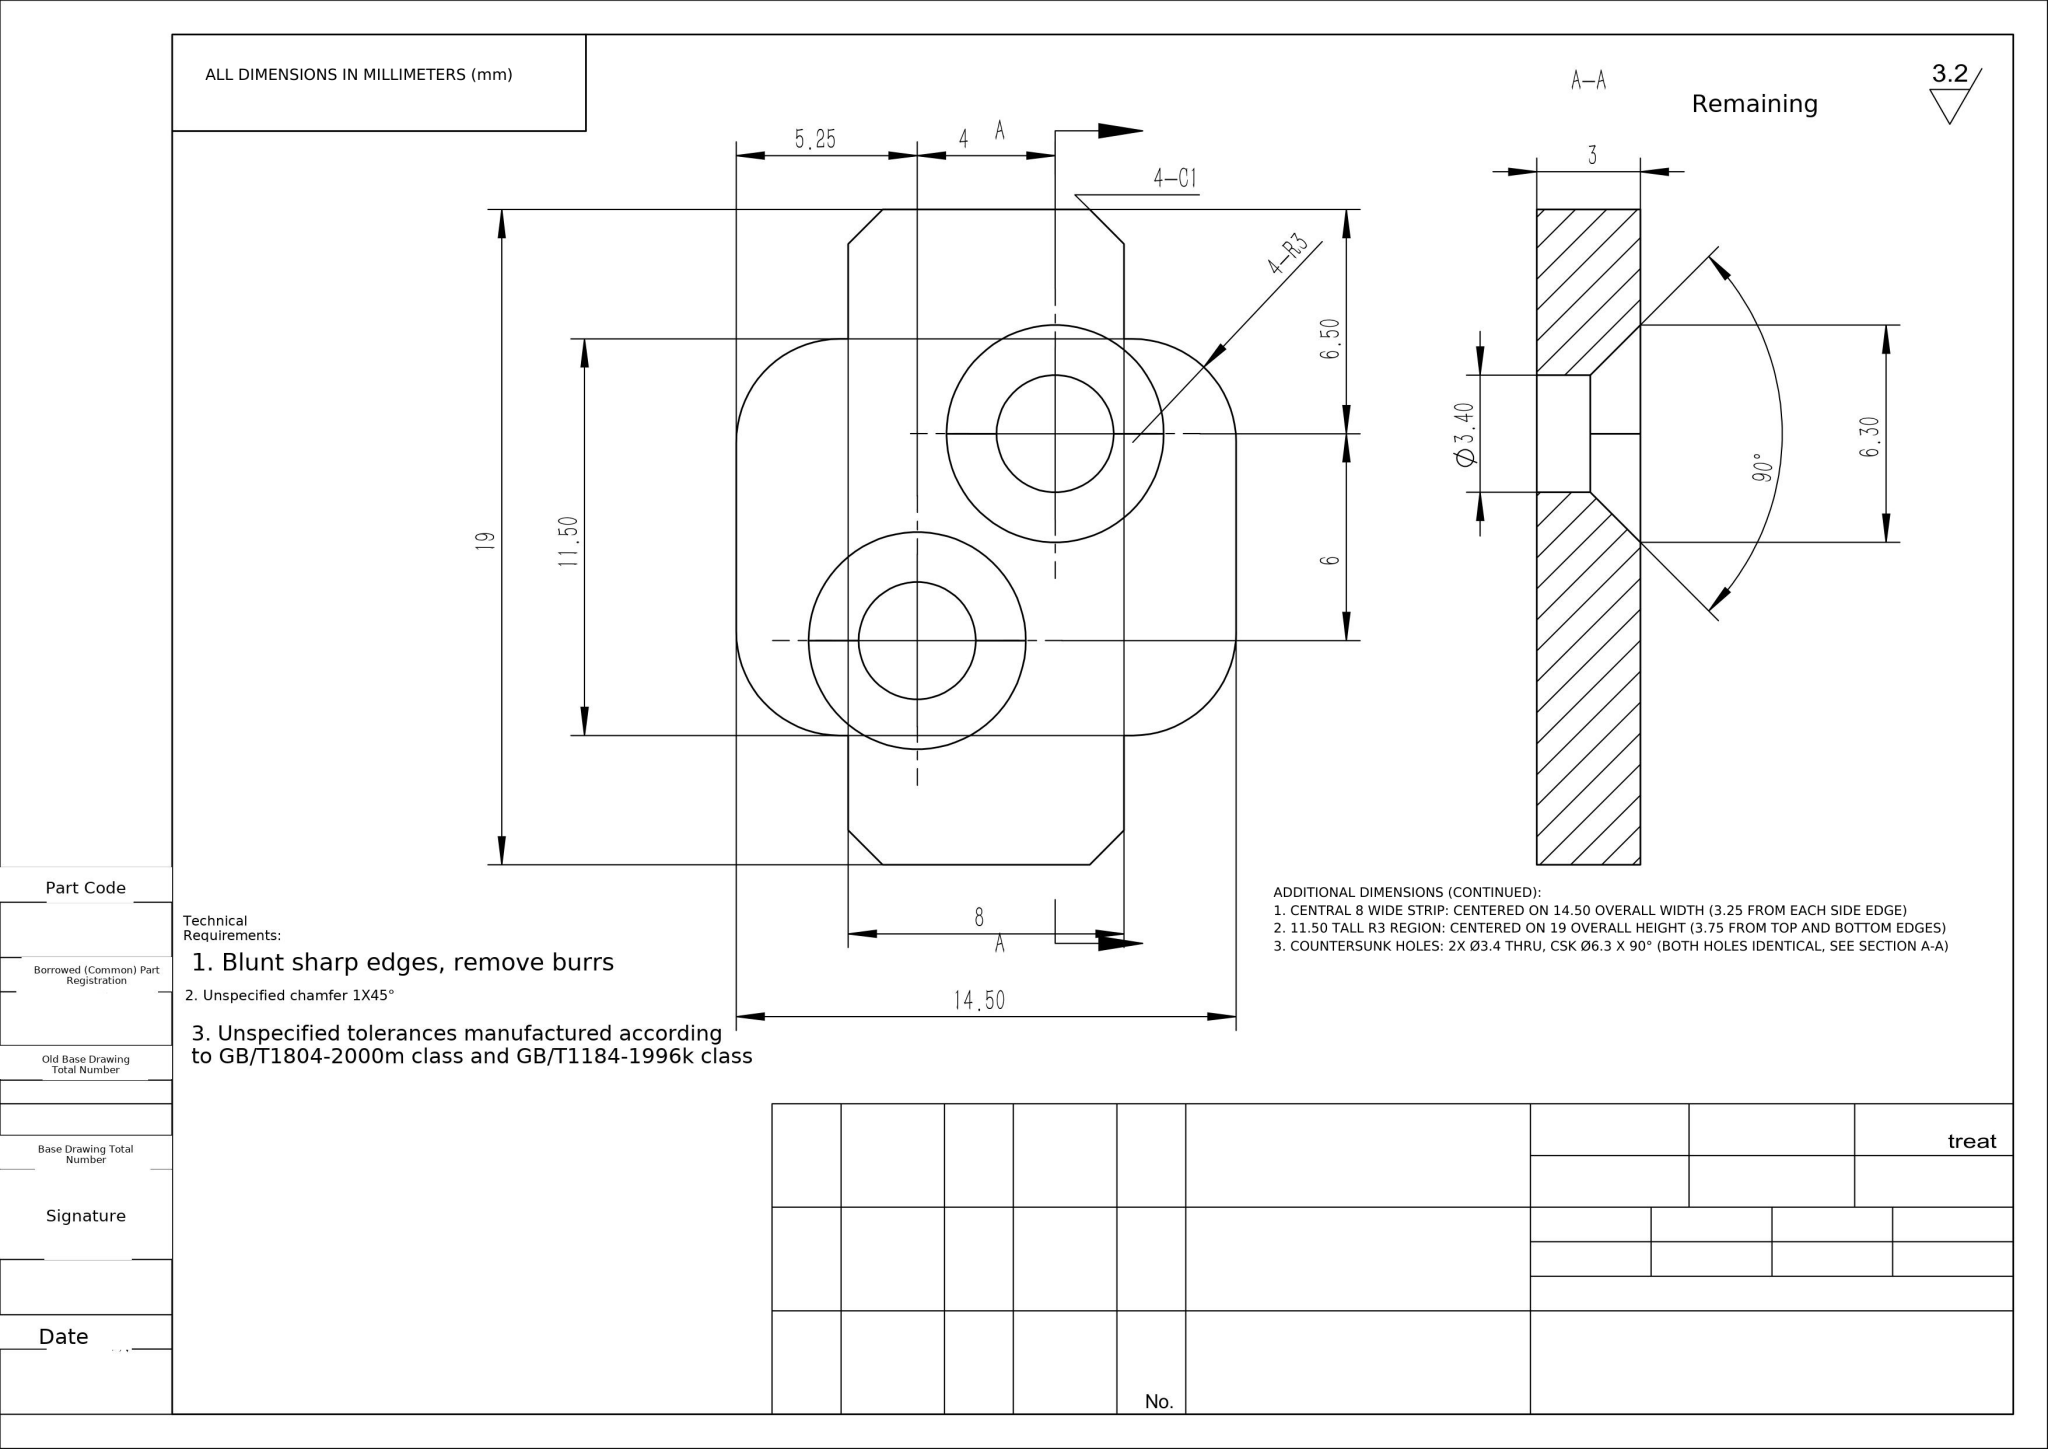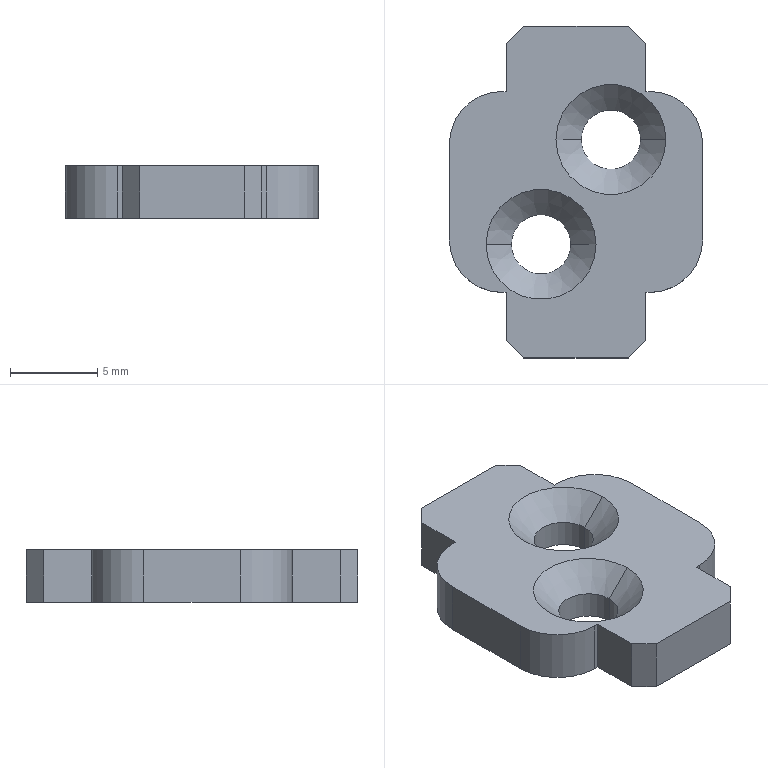Part | NX | mm | 1 solid | 30 faces | box 14.5 x 19 x 3 mm | volume 568 mm3 | plane 18 | cylinder 8 | cone 4 | commonest cylinder face diameters 3.4 x4 6 x4
STEP:
#1=COLOUR_RGB('',1.,1.,1.);
#2=FILL_AREA_STYLE_COLOUR('',#1);
#3=FILL_AREA_STYLE('',(#2));
#4=SURFACE_STYLE_FILL_AREA(#3);
#5=SURFACE_SIDE_STYLE('',(#4));
#6=SURFACE_STYLE_USAGE(.BOTH.,#5);
#7=PRESENTATION_STYLE_ASSIGNMENT((#6));
#8=CARTESIAN_POINT('',(-0.3,-3.,-1.5));
#9=VERTEX_POINT('',#8);
#10=CARTESIAN_POINT('',(-3.7,-3.,-1.5));
#11=VERTEX_POINT('',#10);
#12=CARTESIAN_POINT('',(-2.,-3.,-1.5));
#13=DIRECTION('',(0.,0.,-1.));
#14=DIRECTION('',(1.,0.,0.));
#15=AXIS2_PLACEMENT_3D('',#12,#13,#14);
#16=CIRCLE('',#15,1.7);
#17=EDGE_CURVE('',#9,#11,#16,.T.);
#18=ORIENTED_EDGE('',*,*,#17,.T.);
#19=CARTESIAN_POINT('',(-3.7,-3.,0.05));
#20=VERTEX_POINT('',#19);
#21=CARTESIAN_POINT('',(-3.7,-3.,-22.588));
#22=DIRECTION('',(0.,0.,1.));
#23=VECTOR('',#22,1000.);
#24=LINE('',#21,#23);
#25=EDGE_CURVE('',#11,#20,#24,.T.);
#26=ORIENTED_EDGE('',*,*,#25,.T.);
#27=CARTESIAN_POINT('',(-0.3,-3.,0.05));
#28=VERTEX_POINT('',#27);
#29=CARTESIAN_POINT('',(-2.,-3.,0.05));
#30=DIRECTION('',(0.,0.,-1.));
#31=DIRECTION('',(1.,0.,0.));
#32=AXIS2_PLACEMENT_3D('',#29,#30,#31);
#33=CIRCLE('',#32,1.7);
#34=EDGE_CURVE('',#28,#20,#33,.T.);
#35=ORIENTED_EDGE('',*,*,#34,.F.);
#36=CARTESIAN_POINT('',(-0.3,-3.,-22.588));
#37=DIRECTION('',(0.,0.,1.));
#38=VECTOR('',#37,1000.);
#39=LINE('',#36,#38);
#40=EDGE_CURVE('',#9,#28,#39,.T.);
#41=ORIENTED_EDGE('',*,*,#40,.F.);
#42=EDGE_LOOP('',(#18,#26,#35,#41));
#43=FACE_OUTER_BOUND('',#42,.T.);
#44=CARTESIAN_POINT('',(-2.,-3.,-22.588));
#45=DIRECTION('',(0.,0.,1.));
#46=DIRECTION('',(1.,0.,0.));
#47=AXIS2_PLACEMENT_3D('',#44,#45,#46);
#48=CYLINDRICAL_SURFACE('',#47,1.7);
#49=ADVANCED_FACE('',(#43),#48,.F.);
#50=CARTESIAN_POINT('',(3.7,3.,-1.5));
#51=VERTEX_POINT('',#50);
#52=CARTESIAN_POINT('',(0.3,3.,-1.5));
#53=VERTEX_POINT('',#52);
#54=CARTESIAN_POINT('',(2.,3.,-1.5));
#55=DIRECTION('',(0.,0.,-1.));
#56=DIRECTION('',(1.,0.,0.));
#57=AXIS2_PLACEMENT_3D('',#54,#55,#56);
#58=CIRCLE('',#57,1.7);
#59=EDGE_CURVE('',#51,#53,#58,.T.);
#60=ORIENTED_EDGE('',*,*,#59,.T.);
#61=CARTESIAN_POINT('',(0.3,3.,0.05));
#62=VERTEX_POINT('',#61);
#63=CARTESIAN_POINT('',(0.3,3.,-22.588));
#64=DIRECTION('',(0.,0.,1.));
#65=VECTOR('',#64,1000.);
#66=LINE('',#63,#65);
#67=EDGE_CURVE('',#53,#62,#66,.T.);
#68=ORIENTED_EDGE('',*,*,#67,.T.);
#69=CARTESIAN_POINT('',(3.7,3.,0.05));
#70=VERTEX_POINT('',#69);
#71=CARTESIAN_POINT('',(2.,3.,0.05));
#72=DIRECTION('',(0.,0.,-1.));
#73=DIRECTION('',(1.,0.,0.));
#74=AXIS2_PLACEMENT_3D('',#71,#72,#73);
#75=CIRCLE('',#74,1.7);
#76=EDGE_CURVE('',#70,#62,#75,.T.);
#77=ORIENTED_EDGE('',*,*,#76,.F.);
#78=CARTESIAN_POINT('',(3.7,3.,-22.588));
#79=DIRECTION('',(0.,0.,1.));
#80=VECTOR('',#79,1000.);
#81=LINE('',#78,#80);
#82=EDGE_CURVE('',#51,#70,#81,.T.);
#83=ORIENTED_EDGE('',*,*,#82,.F.);
#84=EDGE_LOOP('',(#60,#68,#77,#83));
#85=FACE_OUTER_BOUND('',#84,.T.);
#86=CARTESIAN_POINT('',(2.,3.,-22.588));
#87=DIRECTION('',(0.,0.,1.));
#88=DIRECTION('',(1.,0.,0.));
#89=AXIS2_PLACEMENT_3D('',#86,#87,#88);
#90=CYLINDRICAL_SURFACE('',#89,1.7);
#91=ADVANCED_FACE('',(#85),#90,.F.);
#92=ORIENTED_EDGE('',*,*,#17,.F.);
#93=CARTESIAN_POINT('',(-2.,-3.,-1.5));
#94=DIRECTION('',(0.,0.,-1.));
#95=DIRECTION('',(1.,0.,0.));
#96=AXIS2_PLACEMENT_3D('',#93,#94,#95);
#97=CIRCLE('',#96,1.7);
#98=EDGE_CURVE('',#11,#9,#97,.T.);
#99=ORIENTED_EDGE('',*,*,#98,.F.);
#100=EDGE_LOOP('',(#92,#99));
#101=FACE_BOUND('',#100,.T.);
#102=ORIENTED_EDGE('',*,*,#59,.F.);
#103=CARTESIAN_POINT('',(2.,3.,-1.5));
#104=DIRECTION('',(0.,0.,-1.));
#105=DIRECTION('',(1.,0.,0.));
#106=AXIS2_PLACEMENT_3D('',#103,#104,#105);
#107=CIRCLE('',#106,1.7);
#108=EDGE_CURVE('',#53,#51,#107,.T.);
#109=ORIENTED_EDGE('',*,*,#108,.F.);
#110=EDGE_LOOP('',(#102,#109));
#111=FACE_BOUND('',#110,.T.);
#112=CARTESIAN_POINT('',(3.,9.5,-1.5));
#113=VERTEX_POINT('',#112);
#114=CARTESIAN_POINT('',(-3.,9.5,-1.5));
#115=VERTEX_POINT('',#114);
#116=CARTESIAN_POINT('',(0.,9.5,-1.5));
#117=DIRECTION('',(-1.,0.,0.));
#118=VECTOR('',#117,1000.);
#119=LINE('',#116,#118);
#120=EDGE_CURVE('',#113,#115,#119,.T.);
#121=ORIENTED_EDGE('',*,*,#120,.F.);
#122=CARTESIAN_POINT('',(4.,8.5,-1.5));
#123=VERTEX_POINT('',#122);
#124=CARTESIAN_POINT('',(3.5,9.,-1.5));
#125=DIRECTION('',(-0.7071,0.7071,0.));
#126=VECTOR('',#125,1000.);
#127=LINE('',#124,#126);
#128=EDGE_CURVE('',#123,#113,#127,.T.);
#129=ORIENTED_EDGE('',*,*,#128,.F.);
#130=CARTESIAN_POINT('',(4.,5.75,-1.5));
#131=VERTEX_POINT('',#130);
#132=CARTESIAN_POINT('',(4.,0.,-1.5));
#133=DIRECTION('',(0.,1.,0.));
#134=VECTOR('',#133,1000.);
#135=LINE('',#132,#134);
#136=EDGE_CURVE('',#131,#123,#135,.T.);
#137=ORIENTED_EDGE('',*,*,#136,.F.);
#138=CARTESIAN_POINT('',(4.25,5.75,-1.5));
#139=VERTEX_POINT('',#138);
#140=CARTESIAN_POINT('',(4.,5.75,-1.5));
#141=DIRECTION('',(1.,0.,0.));
#142=VECTOR('',#141,1000.);
#143=LINE('',#140,#142);
#144=EDGE_CURVE('',#131,#139,#143,.T.);
#145=ORIENTED_EDGE('',*,*,#144,.T.);
#146=CARTESIAN_POINT('',(7.25,2.75,-1.5));
#147=VERTEX_POINT('',#146);
#148=CARTESIAN_POINT('',(4.25,2.75,-1.5));
#149=DIRECTION('',(0.,0.,1.));
#150=DIRECTION('',(1.,0.,0.));
#151=AXIS2_PLACEMENT_3D('',#148,#149,#150);
#152=CIRCLE('',#151,3.);
#153=EDGE_CURVE('',#147,#139,#152,.T.);
#154=ORIENTED_EDGE('',*,*,#153,.F.);
#155=CARTESIAN_POINT('',(7.25,-2.75,-1.5));
#156=VERTEX_POINT('',#155);
#157=CARTESIAN_POINT('',(7.25,0.,-1.5));
#158=DIRECTION('',(0.,1.,0.));
#159=VECTOR('',#158,1000.);
#160=LINE('',#157,#159);
#161=EDGE_CURVE('',#156,#147,#160,.T.);
#162=ORIENTED_EDGE('',*,*,#161,.F.);
#163=CARTESIAN_POINT('',(4.25,-5.75,-1.5));
#164=VERTEX_POINT('',#163);
#165=CARTESIAN_POINT('',(4.25,-2.75,-1.5));
#166=DIRECTION('',(0.,0.,1.));
#167=DIRECTION('',(-1.,0.,0.));
#168=AXIS2_PLACEMENT_3D('',#165,#166,#167);
#169=CIRCLE('',#168,3.);
#170=EDGE_CURVE('',#164,#156,#169,.T.);
#171=ORIENTED_EDGE('',*,*,#170,.F.);
#172=CARTESIAN_POINT('',(4.,-5.75,-1.5));
#173=VERTEX_POINT('',#172);
#174=CARTESIAN_POINT('',(7.25,-5.75,-1.5));
#175=DIRECTION('',(-1.,0.,0.));
#176=VECTOR('',#175,1000.);
#177=LINE('',#174,#176);
#178=EDGE_CURVE('',#164,#173,#177,.T.);
#179=ORIENTED_EDGE('',*,*,#178,.T.);
#180=CARTESIAN_POINT('',(4.,-8.5,-1.5));
#181=VERTEX_POINT('',#180);
#182=CARTESIAN_POINT('',(4.,0.,-1.5));
#183=DIRECTION('',(0.,1.,0.));
#184=VECTOR('',#183,1000.);
#185=LINE('',#182,#184);
#186=EDGE_CURVE('',#181,#173,#185,.T.);
#187=ORIENTED_EDGE('',*,*,#186,.F.);
#188=CARTESIAN_POINT('',(3.,-9.5,-1.5));
#189=VERTEX_POINT('',#188);
#190=CARTESIAN_POINT('',(3.5,-9.,-1.5));
#191=DIRECTION('',(0.7071,0.7071,0.));
#192=VECTOR('',#191,1000.);
#193=LINE('',#190,#192);
#194=EDGE_CURVE('',#189,#181,#193,.T.);
#195=ORIENTED_EDGE('',*,*,#194,.F.);
#196=CARTESIAN_POINT('',(-3.,-9.5,-1.5));
#197=VERTEX_POINT('',#196);
#198=CARTESIAN_POINT('',(0.,-9.5,-1.5));
#199=DIRECTION('',(1.,0.,0.));
#200=VECTOR('',#199,1000.);
#201=LINE('',#198,#200);
#202=EDGE_CURVE('',#197,#189,#201,.T.);
#203=ORIENTED_EDGE('',*,*,#202,.F.);
#204=CARTESIAN_POINT('',(-4.,-8.5,-1.5));
#205=VERTEX_POINT('',#204);
#206=CARTESIAN_POINT('',(-3.5,-9.,-1.5));
#207=DIRECTION('',(0.7071,-0.7071,0.));
#208=VECTOR('',#207,1000.);
#209=LINE('',#206,#208);
#210=EDGE_CURVE('',#205,#197,#209,.T.);
#211=ORIENTED_EDGE('',*,*,#210,.F.);
#212=CARTESIAN_POINT('',(-4.,-5.75,-1.5));
#213=VERTEX_POINT('',#212);
#214=CARTESIAN_POINT('',(-4.,0.,-1.5));
#215=DIRECTION('',(0.,-1.,0.));
#216=VECTOR('',#215,1000.);
#217=LINE('',#214,#216);
#218=EDGE_CURVE('',#213,#205,#217,.T.);
#219=ORIENTED_EDGE('',*,*,#218,.F.);
#220=CARTESIAN_POINT('',(-4.25,-5.75,-1.5));
#221=VERTEX_POINT('',#220);
#222=CARTESIAN_POINT('',(-4.,-5.75,-1.5));
#223=DIRECTION('',(-1.,0.,0.));
#224=VECTOR('',#223,1000.);
#225=LINE('',#222,#224);
#226=EDGE_CURVE('',#213,#221,#225,.T.);
#227=ORIENTED_EDGE('',*,*,#226,.T.);
#228=CARTESIAN_POINT('',(-7.25,-2.75,-1.5));
#229=VERTEX_POINT('',#228);
#230=CARTESIAN_POINT('',(-4.25,-2.75,-1.5));
#231=DIRECTION('',(0.,0.,1.));
#232=DIRECTION('',(1.,0.,0.));
#233=AXIS2_PLACEMENT_3D('',#230,#231,#232);
#234=CIRCLE('',#233,3.);
#235=EDGE_CURVE('',#229,#221,#234,.T.);
#236=ORIENTED_EDGE('',*,*,#235,.F.);
#237=CARTESIAN_POINT('',(-7.25,2.75,-1.5));
#238=VERTEX_POINT('',#237);
#239=CARTESIAN_POINT('',(-7.25,0.,-1.5));
#240=DIRECTION('',(0.,-1.,0.));
#241=VECTOR('',#240,1000.);
#242=LINE('',#239,#241);
#243=EDGE_CURVE('',#238,#229,#242,.T.);
#244=ORIENTED_EDGE('',*,*,#243,.F.);
#245=CARTESIAN_POINT('',(-4.25,5.75,-1.5));
#246=VERTEX_POINT('',#245);
#247=CARTESIAN_POINT('',(-4.25,2.75,-1.5));
#248=DIRECTION('',(0.,0.,1.));
#249=DIRECTION('',(-1.,-0.,0.));
#250=AXIS2_PLACEMENT_3D('',#247,#248,#249);
#251=CIRCLE('',#250,3.);
#252=EDGE_CURVE('',#246,#238,#251,.T.);
#253=ORIENTED_EDGE('',*,*,#252,.F.);
#254=CARTESIAN_POINT('',(-4.,5.75,-1.5));
#255=VERTEX_POINT('',#254);
#256=CARTESIAN_POINT('',(-7.25,5.75,-1.5));
#257=DIRECTION('',(1.,0.,0.));
#258=VECTOR('',#257,1000.);
#259=LINE('',#256,#258);
#260=EDGE_CURVE('',#246,#255,#259,.T.);
#261=ORIENTED_EDGE('',*,*,#260,.T.);
#262=CARTESIAN_POINT('',(-4.,8.5,-1.5));
#263=VERTEX_POINT('',#262);
#264=CARTESIAN_POINT('',(-4.,0.,-1.5));
#265=DIRECTION('',(0.,-1.,0.));
#266=VECTOR('',#265,1000.);
#267=LINE('',#264,#266);
#268=EDGE_CURVE('',#263,#255,#267,.T.);
#269=ORIENTED_EDGE('',*,*,#268,.F.);
#270=CARTESIAN_POINT('',(-3.5,9.,-1.5));
#271=DIRECTION('',(-0.7071,-0.7071,0.));
#272=VECTOR('',#271,1000.);
#273=LINE('',#270,#272);
#274=EDGE_CURVE('',#115,#263,#273,.T.);
#275=ORIENTED_EDGE('',*,*,#274,.F.);
#276=EDGE_LOOP('',(#121,#129,#137,#145,#154,#162,#171,#179,#187,#195,#203,#211,#219,#227,#236,#244,#253,#261,#269,#275));
#277=FACE_OUTER_BOUND('',#276,.T.);
#278=CARTESIAN_POINT('',(0.,0.,-1.5));
#279=DIRECTION('',(0.,0.,1.));
#280=DIRECTION('',(1.,0.,0.));
#281=AXIS2_PLACEMENT_3D('',#278,#279,#280);
#282=PLANE('',#281);
#283=ADVANCED_FACE('',(#101,#111,#277),#282,.F.);
#284=ORIENTED_EDGE('',*,*,#25,.F.);
#285=ORIENTED_EDGE('',*,*,#98,.T.);
#286=ORIENTED_EDGE('',*,*,#40,.T.);
#287=CARTESIAN_POINT('',(-2.,-3.,0.05));
#288=DIRECTION('',(0.,0.,-1.));
#289=DIRECTION('',(1.,0.,0.));
#290=AXIS2_PLACEMENT_3D('',#287,#288,#289);
#291=CIRCLE('',#290,1.7);
#292=EDGE_CURVE('',#20,#28,#291,.T.);
#293=ORIENTED_EDGE('',*,*,#292,.F.);
#294=EDGE_LOOP('',(#284,#285,#286,#293));
#295=FACE_OUTER_BOUND('',#294,.T.);
#296=CARTESIAN_POINT('',(-2.,-3.,-22.588));
#297=DIRECTION('',(0.,0.,1.));
#298=DIRECTION('',(1.,0.,0.));
#299=AXIS2_PLACEMENT_3D('',#296,#297,#298);
#300=CYLINDRICAL_SURFACE('',#299,1.7);
#301=ADVANCED_FACE('',(#295),#300,.F.);
#302=ORIENTED_EDGE('',*,*,#67,.F.);
#303=ORIENTED_EDGE('',*,*,#108,.T.);
#304=ORIENTED_EDGE('',*,*,#82,.T.);
#305=CARTESIAN_POINT('',(2.,3.,0.05));
#306=DIRECTION('',(0.,0.,-1.));
#307=DIRECTION('',(1.,0.,0.));
#308=AXIS2_PLACEMENT_3D('',#305,#306,#307);
#309=CIRCLE('',#308,1.7);
#310=EDGE_CURVE('',#62,#70,#309,.T.);
#311=ORIENTED_EDGE('',*,*,#310,.F.);
#312=EDGE_LOOP('',(#302,#303,#304,#311));
#313=FACE_OUTER_BOUND('',#312,.T.);
#314=CARTESIAN_POINT('',(2.,3.,-22.588));
#315=DIRECTION('',(0.,0.,1.));
#316=DIRECTION('',(1.,0.,0.));
#317=AXIS2_PLACEMENT_3D('',#314,#315,#316);
#318=CYLINDRICAL_SURFACE('',#317,1.7);
#319=ADVANCED_FACE('',(#313),#318,.F.);
#320=CARTESIAN_POINT('',(3.,9.5,1.5));
#321=VERTEX_POINT('',#320);
#322=CARTESIAN_POINT('',(3.,9.5,0.));
#323=DIRECTION('',(0.,0.,-1.));
#324=VECTOR('',#323,1000.);
#325=LINE('',#322,#324);
#326=EDGE_CURVE('',#321,#113,#325,.T.);
#327=ORIENTED_EDGE('',*,*,#326,.T.);
#328=ORIENTED_EDGE('',*,*,#120,.T.);
#329=CARTESIAN_POINT('',(-3.,9.5,1.5));
#330=VERTEX_POINT('',#329);
#331=CARTESIAN_POINT('',(-3.,9.5,0.));
#332=DIRECTION('',(0.,0.,1.));
#333=VECTOR('',#332,1000.);
#334=LINE('',#331,#333);
#335=EDGE_CURVE('',#115,#330,#334,.T.);
#336=ORIENTED_EDGE('',*,*,#335,.T.);
#337=CARTESIAN_POINT('',(-7.25,9.5,1.5));
#338=DIRECTION('',(1.,0.,0.));
#339=VECTOR('',#338,1000.);
#340=LINE('',#337,#339);
#341=EDGE_CURVE('',#330,#321,#340,.T.);
#342=ORIENTED_EDGE('',*,*,#341,.T.);
#343=EDGE_LOOP('',(#327,#328,#336,#342));
#344=FACE_OUTER_BOUND('',#343,.T.);
#345=CARTESIAN_POINT('',(-7.25,9.5,0.));
#346=DIRECTION('',(0.,1.,0.));
#347=DIRECTION('',(0.,0.,1.));
#348=AXIS2_PLACEMENT_3D('',#345,#346,#347);
#349=PLANE('',#348);
#350=ADVANCED_FACE('',(#344),#349,.T.);
#351=CARTESIAN_POINT('',(4.,5.75,1.5));
#352=VERTEX_POINT('',#351);
#353=CARTESIAN_POINT('',(4.,8.5,1.5));
#354=VERTEX_POINT('',#353);
#355=CARTESIAN_POINT('',(4.,9.5,1.5));
#356=DIRECTION('',(0.,1.,0.));
#357=VECTOR('',#356,1000.);
#358=LINE('',#355,#357);
#359=EDGE_CURVE('',#352,#354,#358,.T.);
#360=ORIENTED_EDGE('',*,*,#359,.F.);
#361=CARTESIAN_POINT('',(4.,5.75,1.5));
#362=DIRECTION('',(0.,0.,1.));
#363=VECTOR('',#362,1000.);
#364=LINE('',#361,#363);
#365=EDGE_CURVE('',#131,#352,#364,.T.);
#366=ORIENTED_EDGE('',*,*,#365,.F.);
#367=ORIENTED_EDGE('',*,*,#136,.T.);
#368=CARTESIAN_POINT('',(4.,8.5,1.5));
#369=DIRECTION('',(0.,0.,-1.));
#370=VECTOR('',#369,1000.);
#371=LINE('',#368,#370);
#372=EDGE_CURVE('',#354,#123,#371,.T.);
#373=ORIENTED_EDGE('',*,*,#372,.F.);
#374=EDGE_LOOP('',(#360,#366,#367,#373));
#375=FACE_OUTER_BOUND('',#374,.T.);
#376=CARTESIAN_POINT('',(4.,9.5,1.5));
#377=DIRECTION('',(-1.,0.,0.));
#378=DIRECTION('',(0.,0.,1.));
#379=AXIS2_PLACEMENT_3D('',#376,#377,#378);
#380=PLANE('',#379);
#381=ADVANCED_FACE('',(#375),#380,.F.);
#382=CARTESIAN_POINT('',(4.25,5.75,1.5));
#383=VERTEX_POINT('',#382);
#384=CARTESIAN_POINT('',(4.25,5.75,0.75));
#385=DIRECTION('',(0.,0.,1.));
#386=VECTOR('',#385,1000.);
#387=LINE('',#384,#386);
#388=EDGE_CURVE('',#139,#383,#387,.T.);
#389=ORIENTED_EDGE('',*,*,#388,.T.);
#390=CARTESIAN_POINT('',(7.25,2.75,1.5));
#391=VERTEX_POINT('',#390);
#392=CARTESIAN_POINT('',(4.25,2.75,1.5));
#393=DIRECTION('',(0.,0.,-1.));
#394=DIRECTION('',(1.,0.,0.));
#395=AXIS2_PLACEMENT_3D('',#392,#393,#394);
#396=CIRCLE('',#395,3.);
#397=EDGE_CURVE('',#383,#391,#396,.T.);
#398=ORIENTED_EDGE('',*,*,#397,.T.);
#399=CARTESIAN_POINT('',(7.25,2.75,0.75));
#400=DIRECTION('',(0.,0.,-1.));
#401=VECTOR('',#400,1000.);
#402=LINE('',#399,#401);
#403=EDGE_CURVE('',#391,#147,#402,.T.);
#404=ORIENTED_EDGE('',*,*,#403,.T.);
#405=ORIENTED_EDGE('',*,*,#153,.T.);
#406=EDGE_LOOP('',(#389,#398,#404,#405));
#407=FACE_OUTER_BOUND('',#406,.T.);
#408=CARTESIAN_POINT('',(4.25,2.75,0.75));
#409=DIRECTION('',(0.,0.,1.));
#410=DIRECTION('',(1.,0.,0.));
#411=AXIS2_PLACEMENT_3D('',#408,#409,#410);
#412=CYLINDRICAL_SURFACE('',#411,3.);
#413=ADVANCED_FACE('',(#407),#412,.T.);
#414=CARTESIAN_POINT('',(7.25,-2.75,1.5));
#415=VERTEX_POINT('',#414);
#416=CARTESIAN_POINT('',(7.25,-2.75,0.));
#417=DIRECTION('',(0.,0.,-1.));
#418=VECTOR('',#417,1000.);
#419=LINE('',#416,#418);
#420=EDGE_CURVE('',#415,#156,#419,.T.);
#421=ORIENTED_EDGE('',*,*,#420,.T.);
#422=ORIENTED_EDGE('',*,*,#161,.T.);
#423=ORIENTED_EDGE('',*,*,#403,.F.);
#424=CARTESIAN_POINT('',(7.25,9.5,1.5));
#425=DIRECTION('',(0.,-1.,0.));
#426=VECTOR('',#425,1000.);
#427=LINE('',#424,#426);
#428=EDGE_CURVE('',#391,#415,#427,.T.);
#429=ORIENTED_EDGE('',*,*,#428,.T.);
#430=EDGE_LOOP('',(#421,#422,#423,#429));
#431=FACE_OUTER_BOUND('',#430,.T.);
#432=CARTESIAN_POINT('',(7.25,9.5,0.));
#433=DIRECTION('',(1.,0.,0.));
#434=DIRECTION('',(0.,0.,-1.));
#435=AXIS2_PLACEMENT_3D('',#432,#433,#434);
#436=PLANE('',#435);
#437=ADVANCED_FACE('',(#431),#436,.T.);
#438=ORIENTED_EDGE('',*,*,#420,.F.);
#439=CARTESIAN_POINT('',(4.25,-5.75,1.5));
#440=VERTEX_POINT('',#439);
#441=CARTESIAN_POINT('',(4.25,-2.75,1.5));
#442=DIRECTION('',(0.,0.,-1.));
#443=DIRECTION('',(-1.,0.,0.));
#444=AXIS2_PLACEMENT_3D('',#441,#442,#443);
#445=CIRCLE('',#444,3.);
#446=EDGE_CURVE('',#415,#440,#445,.T.);
#447=ORIENTED_EDGE('',*,*,#446,.T.);
#448=CARTESIAN_POINT('',(4.25,-5.75,0.75));
#449=DIRECTION('',(0.,0.,-1.));
#450=VECTOR('',#449,1000.);
#451=LINE('',#448,#450);
#452=EDGE_CURVE('',#440,#164,#451,.T.);
#453=ORIENTED_EDGE('',*,*,#452,.T.);
#454=ORIENTED_EDGE('',*,*,#170,.T.);
#455=EDGE_LOOP('',(#438,#447,#453,#454));
#456=FACE_OUTER_BOUND('',#455,.T.);
#457=CARTESIAN_POINT('',(4.25,-2.75,0.75));
#458=DIRECTION('',(0.,0.,-1.));
#459=DIRECTION('',(-1.,0.,0.));
#460=AXIS2_PLACEMENT_3D('',#457,#458,#459);
#461=CYLINDRICAL_SURFACE('',#460,3.);
#462=ADVANCED_FACE('',(#456),#461,.T.);
#463=ORIENTED_EDGE('',*,*,#186,.T.);
#464=CARTESIAN_POINT('',(4.,-5.75,1.5));
#465=VERTEX_POINT('',#464);
#466=CARTESIAN_POINT('',(4.,-5.75,1.5));
#467=DIRECTION('',(0.,0.,-1.));
#468=VECTOR('',#467,1000.);
#469=LINE('',#466,#468);
#470=EDGE_CURVE('',#465,#173,#469,.T.);
#471=ORIENTED_EDGE('',*,*,#470,.F.);
#472=CARTESIAN_POINT('',(4.,-8.5,1.5));
#473=VERTEX_POINT('',#472);
#474=CARTESIAN_POINT('',(4.,-5.75,1.5));
#475=DIRECTION('',(0.,1.,0.));
#476=VECTOR('',#475,1000.);
#477=LINE('',#474,#476);
#478=EDGE_CURVE('',#473,#465,#477,.T.);
#479=ORIENTED_EDGE('',*,*,#478,.F.);
#480=CARTESIAN_POINT('',(4.,-8.5,1.5));
#481=DIRECTION('',(0.,0.,1.));
#482=VECTOR('',#481,1000.);
#483=LINE('',#480,#482);
#484=EDGE_CURVE('',#181,#473,#483,.T.);
#485=ORIENTED_EDGE('',*,*,#484,.F.);
#486=EDGE_LOOP('',(#463,#471,#479,#485));
#487=FACE_OUTER_BOUND('',#486,.T.);
#488=CARTESIAN_POINT('',(4.,-5.75,1.5));
#489=DIRECTION('',(-1.,0.,0.));
#490=DIRECTION('',(0.,0.,1.));
#491=AXIS2_PLACEMENT_3D('',#488,#489,#490);
#492=PLANE('',#491);
#493=ADVANCED_FACE('',(#487),#492,.F.);
#494=CARTESIAN_POINT('',(-3.,-9.5,1.5));
#495=VERTEX_POINT('',#494);
#496=CARTESIAN_POINT('',(-3.,-9.5,0.));
#497=DIRECTION('',(0.,0.,-1.));
#498=VECTOR('',#497,1000.);
#499=LINE('',#496,#498);
#500=EDGE_CURVE('',#495,#197,#499,.T.);
#501=ORIENTED_EDGE('',*,*,#500,.T.);
#502=ORIENTED_EDGE('',*,*,#202,.T.);
#503=CARTESIAN_POINT('',(3.,-9.5,1.5));
#504=VERTEX_POINT('',#503);
#505=CARTESIAN_POINT('',(3.,-9.5,0.));
#506=DIRECTION('',(0.,0.,1.));
#507=VECTOR('',#506,1000.);
#508=LINE('',#505,#507);
#509=EDGE_CURVE('',#189,#504,#508,.T.);
#510=ORIENTED_EDGE('',*,*,#509,.T.);
#511=CARTESIAN_POINT('',(7.25,-9.5,1.5));
#512=DIRECTION('',(-1.,0.,0.));
#513=VECTOR('',#512,1000.);
#514=LINE('',#511,#513);
#515=EDGE_CURVE('',#504,#495,#514,.T.);
#516=ORIENTED_EDGE('',*,*,#515,.T.);
#517=EDGE_LOOP('',(#501,#502,#510,#516));
#518=FACE_OUTER_BOUND('',#517,.T.);
#519=CARTESIAN_POINT('',(7.25,-9.5,0.));
#520=DIRECTION('',(0.,-1.,0.));
#521=DIRECTION('',(0.,0.,-1.));
#522=AXIS2_PLACEMENT_3D('',#519,#520,#521);
#523=PLANE('',#522);
#524=ADVANCED_FACE('',(#518),#523,.T.);
#525=CARTESIAN_POINT('',(-4.,-5.75,1.5));
#526=VERTEX_POINT('',#525);
#527=CARTESIAN_POINT('',(-4.,-8.5,1.5));
#528=VERTEX_POINT('',#527);
#529=CARTESIAN_POINT('',(-4.,-9.5,1.5));
#530=DIRECTION('',(0.,-1.,0.));
#531=VECTOR('',#530,1000.);
#532=LINE('',#529,#531);
#533=EDGE_CURVE('',#526,#528,#532,.T.);
#534=ORIENTED_EDGE('',*,*,#533,.F.);
#535=CARTESIAN_POINT('',(-4.,-5.75,1.5));
#536=DIRECTION('',(0.,0.,1.));
#537=VECTOR('',#536,1000.);
#538=LINE('',#535,#537);
#539=EDGE_CURVE('',#213,#526,#538,.T.);
#540=ORIENTED_EDGE('',*,*,#539,.F.);
#541=ORIENTED_EDGE('',*,*,#218,.T.);
#542=CARTESIAN_POINT('',(-4.,-8.5,1.5));
#543=DIRECTION('',(0.,0.,-1.));
#544=VECTOR('',#543,1000.);
#545=LINE('',#542,#544);
#546=EDGE_CURVE('',#528,#205,#545,.T.);
#547=ORIENTED_EDGE('',*,*,#546,.F.);
#548=EDGE_LOOP('',(#534,#540,#541,#547));
#549=FACE_OUTER_BOUND('',#548,.T.);
#550=CARTESIAN_POINT('',(-4.,-9.5,1.5));
#551=DIRECTION('',(1.,0.,0.));
#552=DIRECTION('',(0.,0.,-1.));
#553=AXIS2_PLACEMENT_3D('',#550,#551,#552);
#554=PLANE('',#553);
#555=ADVANCED_FACE('',(#549),#554,.F.);
#556=CARTESIAN_POINT('',(-4.25,-5.75,1.5));
#557=VERTEX_POINT('',#556);
#558=CARTESIAN_POINT('',(-4.25,-5.75,0.75));
#559=DIRECTION('',(0.,0.,1.));
#560=VECTOR('',#559,1000.);
#561=LINE('',#558,#560);
#562=EDGE_CURVE('',#221,#557,#561,.T.);
#563=ORIENTED_EDGE('',*,*,#562,.T.);
#564=CARTESIAN_POINT('',(-7.25,-2.75,1.5));
#565=VERTEX_POINT('',#564);
#566=CARTESIAN_POINT('',(-4.25,-2.75,1.5));
#567=DIRECTION('',(0.,0.,-1.));
#568=DIRECTION('',(1.,0.,0.));
#569=AXIS2_PLACEMENT_3D('',#566,#567,#568);
#570=CIRCLE('',#569,3.);
#571=EDGE_CURVE('',#557,#565,#570,.T.);
#572=ORIENTED_EDGE('',*,*,#571,.T.);
#573=CARTESIAN_POINT('',(-7.25,-2.75,0.75));
#574=DIRECTION('',(0.,0.,-1.));
#575=VECTOR('',#574,1000.);
#576=LINE('',#573,#575);
#577=EDGE_CURVE('',#565,#229,#576,.T.);
#578=ORIENTED_EDGE('',*,*,#577,.T.);
#579=ORIENTED_EDGE('',*,*,#235,.T.);
#580=EDGE_LOOP('',(#563,#572,#578,#579));
#581=FACE_OUTER_BOUND('',#580,.T.);
#582=CARTESIAN_POINT('',(-4.25,-2.75,0.75));
#583=DIRECTION('',(0.,0.,1.));
#584=DIRECTION('',(1.,0.,0.));
#585=AXIS2_PLACEMENT_3D('',#582,#583,#584);
#586=CYLINDRICAL_SURFACE('',#585,3.);
#587=ADVANCED_FACE('',(#581),#586,.T.);
#588=ORIENTED_EDGE('',*,*,#577,.F.);
#589=CARTESIAN_POINT('',(-7.25,2.75,1.5));
#590=VERTEX_POINT('',#589);
#591=CARTESIAN_POINT('',(-7.25,-9.5,1.5));
#592=DIRECTION('',(0.,1.,0.));
#593=VECTOR('',#592,1000.);
#594=LINE('',#591,#593);
#595=EDGE_CURVE('',#565,#590,#594,.T.);
#596=ORIENTED_EDGE('',*,*,#595,.T.);
#597=CARTESIAN_POINT('',(-7.25,2.75,0.));
#598=DIRECTION('',(0.,0.,-1.));
#599=VECTOR('',#598,1000.);
#600=LINE('',#597,#599);
#601=EDGE_CURVE('',#590,#238,#600,.T.);
#602=ORIENTED_EDGE('',*,*,#601,.T.);
#603=ORIENTED_EDGE('',*,*,#243,.T.);
#604=EDGE_LOOP('',(#588,#596,#602,#603));
#605=FACE_OUTER_BOUND('',#604,.T.);
#606=CARTESIAN_POINT('',(-7.25,-9.5,0.));
#607=DIRECTION('',(-1.,0.,0.));
#608=DIRECTION('',(0.,0.,1.));
#609=AXIS2_PLACEMENT_3D('',#606,#607,#608);
#610=PLANE('',#609);
#611=ADVANCED_FACE('',(#605),#610,.T.);
#612=ORIENTED_EDGE('',*,*,#601,.F.);
#613=CARTESIAN_POINT('',(-4.25,5.75,1.5));
#614=VERTEX_POINT('',#613);
#615=CARTESIAN_POINT('',(-4.25,2.75,1.5));
#616=DIRECTION('',(0.,0.,-1.));
#617=DIRECTION('',(-1.,0.,0.));
#618=AXIS2_PLACEMENT_3D('',#615,#616,#617);
#619=CIRCLE('',#618,3.);
#620=EDGE_CURVE('',#590,#614,#619,.T.);
#621=ORIENTED_EDGE('',*,*,#620,.T.);
#622=CARTESIAN_POINT('',(-4.25,5.75,0.75));
#623=DIRECTION('',(0.,0.,-1.));
#624=VECTOR('',#623,1000.);
#625=LINE('',#622,#624);
#626=EDGE_CURVE('',#614,#246,#625,.T.);
#627=ORIENTED_EDGE('',*,*,#626,.T.);
#628=ORIENTED_EDGE('',*,*,#252,.T.);
#629=EDGE_LOOP('',(#612,#621,#627,#628));
#630=FACE_OUTER_BOUND('',#629,.T.);
#631=CARTESIAN_POINT('',(-4.25,2.75,0.75));
#632=DIRECTION('',(0.,0.,-1.));
#633=DIRECTION('',(-1.,0.,0.));
#634=AXIS2_PLACEMENT_3D('',#631,#632,#633);
#635=CYLINDRICAL_SURFACE('',#634,3.);
#636=ADVANCED_FACE('',(#630),#635,.T.);
#637=ORIENTED_EDGE('',*,*,#268,.T.);
#638=CARTESIAN_POINT('',(-4.,5.75,1.5));
#639=VERTEX_POINT('',#638);
#640=CARTESIAN_POINT('',(-4.,5.75,1.5));
#641=DIRECTION('',(0.,0.,-1.));
#642=VECTOR('',#641,1000.);
#643=LINE('',#640,#642);
#644=EDGE_CURVE('',#639,#255,#643,.T.);
#645=ORIENTED_EDGE('',*,*,#644,.F.);
#646=CARTESIAN_POINT('',(-4.,8.5,1.5));
#647=VERTEX_POINT('',#646);
#648=CARTESIAN_POINT('',(-4.,5.75,1.5));
#649=DIRECTION('',(0.,-1.,0.));
#650=VECTOR('',#649,1000.);
#651=LINE('',#648,#650);
#652=EDGE_CURVE('',#647,#639,#651,.T.);
#653=ORIENTED_EDGE('',*,*,#652,.F.);
#654=CARTESIAN_POINT('',(-4.,8.5,1.5));
#655=DIRECTION('',(0.,0.,1.));
#656=VECTOR('',#655,1000.);
#657=LINE('',#654,#656);
#658=EDGE_CURVE('',#263,#647,#657,.T.);
#659=ORIENTED_EDGE('',*,*,#658,.F.);
#660=EDGE_LOOP('',(#637,#645,#653,#659));
#661=FACE_OUTER_BOUND('',#660,.T.);
#662=CARTESIAN_POINT('',(-4.,5.75,1.5));
#663=DIRECTION('',(1.,0.,0.));
#664=DIRECTION('',(0.,0.,-1.));
#665=AXIS2_PLACEMENT_3D('',#662,#663,#664);
#666=PLANE('',#665);
#667=ADVANCED_FACE('',(#661),#666,.F.);
#668=CARTESIAN_POINT('',(-5.15,-3.,1.5));
#669=VERTEX_POINT('',#668);
#670=CARTESIAN_POINT('',(-499003.649,-3.,499000.));
#671=DIRECTION('',(-0.7071,0.,0.7071));
#672=VECTOR('',#671,1000.);
#673=LINE('',#670,#672);
#674=EDGE_CURVE('',#20,#669,#673,.T.);
#675=ORIENTED_EDGE('',*,*,#674,.F.);
#676=ORIENTED_EDGE('',*,*,#292,.T.);
#677=CARTESIAN_POINT('',(1.15,-3.,1.5));
#678=VERTEX_POINT('',#677);
#679=CARTESIAN_POINT('',(498999.649,-3.,499000.));
#680=DIRECTION('',(-0.7071,0.,-0.7071));
#681=VECTOR('',#680,1000.);
#682=LINE('',#679,#681);
#683=EDGE_CURVE('',#678,#28,#682,.T.);
#684=ORIENTED_EDGE('',*,*,#683,.F.);
#685=CARTESIAN_POINT('',(-2.,-3.,1.5));
#686=DIRECTION('',(0.,0.,-1.));
#687=DIRECTION('',(1.,0.,0.));
#688=AXIS2_PLACEMENT_3D('',#685,#686,#687);
#689=CIRCLE('',#688,3.15);
#690=EDGE_CURVE('',#669,#678,#689,.T.);
#691=ORIENTED_EDGE('',*,*,#690,.F.);
#692=EDGE_LOOP('',(#675,#676,#684,#691));
#693=FACE_OUTER_BOUND('',#692,.T.);
#694=CARTESIAN_POINT('',(-2.,-3.,1.5));
#695=DIRECTION('',(0.,0.,1.));
#696=DIRECTION('',(1.,0.,0.));
#697=AXIS2_PLACEMENT_3D('',#694,#695,#696);
#698=CONICAL_SURFACE('',#697,3.15,0.7854);
#699=ADVANCED_FACE('',(#693),#698,.F.);
#700=ORIENTED_EDGE('',*,*,#683,.T.);
#701=ORIENTED_EDGE('',*,*,#34,.T.);
#702=ORIENTED_EDGE('',*,*,#674,.T.);
#703=CARTESIAN_POINT('',(-2.,-3.,1.5));
#704=DIRECTION('',(0.,0.,-1.));
#705=DIRECTION('',(1.,0.,0.));
#706=AXIS2_PLACEMENT_3D('',#703,#704,#705);
#707=CIRCLE('',#706,3.15);
#708=EDGE_CURVE('',#678,#669,#707,.T.);
#709=ORIENTED_EDGE('',*,*,#708,.F.);
#710=EDGE_LOOP('',(#700,#701,#702,#709));
#711=FACE_OUTER_BOUND('',#710,.T.);
#712=CARTESIAN_POINT('',(-2.,-3.,1.5));
#713=DIRECTION('',(0.,0.,1.));
#714=DIRECTION('',(1.,0.,0.));
#715=AXIS2_PLACEMENT_3D('',#712,#713,#714);
#716=CONICAL_SURFACE('',#715,3.15,0.7854);
#717=ADVANCED_FACE('',(#711),#716,.F.);
#718=CARTESIAN_POINT('',(-1.15,3.,1.5));
#719=VERTEX_POINT('',#718);
#720=CARTESIAN_POINT('',(-498996.,3.,498996.351));
#721=DIRECTION('',(-0.7071,0.,0.7071));
#722=VECTOR('',#721,1000.);
#723=LINE('',#720,#722);
#724=EDGE_CURVE('',#62,#719,#723,.T.);
#725=ORIENTED_EDGE('',*,*,#724,.F.);
#726=ORIENTED_EDGE('',*,*,#310,.T.);
#727=CARTESIAN_POINT('',(5.15,3.,1.5));
#728=VERTEX_POINT('',#727);
#729=CARTESIAN_POINT('',(499000.,3.,498996.351));
#730=DIRECTION('',(-0.7071,0.,-0.7071));
#731=VECTOR('',#730,1000.);
#732=LINE('',#729,#731);
#733=EDGE_CURVE('',#728,#70,#732,.T.);
#734=ORIENTED_EDGE('',*,*,#733,.F.);
#735=CARTESIAN_POINT('',(2.,3.,1.5));
#736=DIRECTION('',(0.,0.,-1.));
#737=DIRECTION('',(1.,0.,0.));
#738=AXIS2_PLACEMENT_3D('',#735,#736,#737);
#739=CIRCLE('',#738,3.15);
#740=EDGE_CURVE('',#719,#728,#739,.T.);
#741=ORIENTED_EDGE('',*,*,#740,.F.);
#742=EDGE_LOOP('',(#725,#726,#734,#741));
#743=FACE_OUTER_BOUND('',#742,.T.);
#744=CARTESIAN_POINT('',(2.,3.,1.5));
#745=DIRECTION('',(0.,0.,1.));
#746=DIRECTION('',(1.,0.,0.));
#747=AXIS2_PLACEMENT_3D('',#744,#745,#746);
#748=CONICAL_SURFACE('',#747,3.15,0.7854);
#749=ADVANCED_FACE('',(#743),#748,.F.);
#750=ORIENTED_EDGE('',*,*,#733,.T.);
#751=ORIENTED_EDGE('',*,*,#76,.T.);
#752=ORIENTED_EDGE('',*,*,#724,.T.);
#753=CARTESIAN_POINT('',(2.,3.,1.5));
#754=DIRECTION('',(0.,0.,-1.));
#755=DIRECTION('',(1.,0.,0.));
#756=AXIS2_PLACEMENT_3D('',#753,#754,#755);
#757=CIRCLE('',#756,3.15);
#758=EDGE_CURVE('',#728,#719,#757,.T.);
#759=ORIENTED_EDGE('',*,*,#758,.F.);
#760=EDGE_LOOP('',(#750,#751,#752,#759));
#761=FACE_OUTER_BOUND('',#760,.T.);
#762=CARTESIAN_POINT('',(2.,3.,1.5));
#763=DIRECTION('',(0.,0.,1.));
#764=DIRECTION('',(1.,0.,0.));
#765=AXIS2_PLACEMENT_3D('',#762,#763,#764);
#766=CONICAL_SURFACE('',#765,3.15,0.7854);
#767=ADVANCED_FACE('',(#761),#766,.F.);
#768=CARTESIAN_POINT('',(3.5,9.,1.5));
#769=DIRECTION('',(0.7071,-0.7071,0.));
#770=VECTOR('',#769,1000.);
#771=LINE('',#768,#770);
#772=EDGE_CURVE('',#321,#354,#771,.T.);
#773=ORIENTED_EDGE('',*,*,#772,.T.);
#774=ORIENTED_EDGE('',*,*,#372,.T.);
#775=ORIENTED_EDGE('',*,*,#128,.T.);
#776=ORIENTED_EDGE('',*,*,#326,.F.);
#777=EDGE_LOOP('',(#773,#774,#775,#776));
#778=FACE_OUTER_BOUND('',#777,.T.);
#779=CARTESIAN_POINT('',(3.5,9.,0.75));
#780=DIRECTION('',(0.7071,0.7071,0.));
#781=DIRECTION('',(-0.7071,0.7071,0.));
#782=AXIS2_PLACEMENT_3D('',#779,#780,#781);
#783=PLANE('',#782);
#784=ADVANCED_FACE('',(#778),#783,.T.);
#785=ORIENTED_EDGE('',*,*,#708,.T.);
#786=ORIENTED_EDGE('',*,*,#690,.T.);
#787=EDGE_LOOP('',(#785,#786));
#788=FACE_BOUND('',#787,.T.);
#789=ORIENTED_EDGE('',*,*,#758,.T.);
#790=ORIENTED_EDGE('',*,*,#740,.T.);
#791=EDGE_LOOP('',(#789,#790));
#792=FACE_BOUND('',#791,.T.);
#793=ORIENTED_EDGE('',*,*,#772,.F.);
#794=ORIENTED_EDGE('',*,*,#341,.F.);
#795=CARTESIAN_POINT('',(-3.,9.5,1.5));
#796=DIRECTION('',(-0.7071,-0.7071,0.));
#797=VECTOR('',#796,1000.);
#798=LINE('',#795,#797);
#799=EDGE_CURVE('',#330,#647,#798,.T.);
#800=ORIENTED_EDGE('',*,*,#799,.T.);
#801=ORIENTED_EDGE('',*,*,#652,.T.);
#802=CARTESIAN_POINT('',(0.,5.75,1.5));
#803=DIRECTION('',(-1.,0.,0.));
#804=VECTOR('',#803,1000.);
#805=LINE('',#802,#804);
#806=EDGE_CURVE('',#639,#614,#805,.T.);
#807=ORIENTED_EDGE('',*,*,#806,.T.);
#808=ORIENTED_EDGE('',*,*,#620,.F.);
#809=ORIENTED_EDGE('',*,*,#595,.F.);
#810=ORIENTED_EDGE('',*,*,#571,.F.);
#811=CARTESIAN_POINT('',(0.,-5.75,1.5));
#812=DIRECTION('',(1.,0.,0.));
#813=VECTOR('',#812,1000.);
#814=LINE('',#811,#813);
#815=EDGE_CURVE('',#557,#526,#814,.T.);
#816=ORIENTED_EDGE('',*,*,#815,.T.);
#817=ORIENTED_EDGE('',*,*,#533,.T.);
#818=CARTESIAN_POINT('',(-4.,-8.5,1.5));
#819=DIRECTION('',(0.7071,-0.7071,0.));
#820=VECTOR('',#819,1000.);
#821=LINE('',#818,#820);
#822=EDGE_CURVE('',#528,#495,#821,.T.);
#823=ORIENTED_EDGE('',*,*,#822,.T.);
#824=ORIENTED_EDGE('',*,*,#515,.F.);
#825=CARTESIAN_POINT('',(3.,-9.5,1.5));
#826=DIRECTION('',(0.7071,0.7071,0.));
#827=VECTOR('',#826,1000.);
#828=LINE('',#825,#827);
#829=EDGE_CURVE('',#504,#473,#828,.T.);
#830=ORIENTED_EDGE('',*,*,#829,.T.);
#831=ORIENTED_EDGE('',*,*,#478,.T.);
#832=CARTESIAN_POINT('',(0.,-5.75,1.5));
#833=DIRECTION('',(1.,0.,0.));
#834=VECTOR('',#833,1000.);
#835=LINE('',#832,#834);
#836=EDGE_CURVE('',#465,#440,#835,.T.);
#837=ORIENTED_EDGE('',*,*,#836,.T.);
#838=ORIENTED_EDGE('',*,*,#446,.F.);
#839=ORIENTED_EDGE('',*,*,#428,.F.);
#840=ORIENTED_EDGE('',*,*,#397,.F.);
#841=CARTESIAN_POINT('',(0.,5.75,1.5));
#842=DIRECTION('',(-1.,0.,0.));
#843=VECTOR('',#842,1000.);
#844=LINE('',#841,#843);
#845=EDGE_CURVE('',#383,#352,#844,.T.);
#846=ORIENTED_EDGE('',*,*,#845,.T.);
#847=ORIENTED_EDGE('',*,*,#359,.T.);
#848=EDGE_LOOP('',(#793,#794,#800,#801,#807,#808,#809,#810,#816,#817,#823,#824,#830,#831,#837,#838,#839,#840,#846,#847));
#849=FACE_OUTER_BOUND('',#848,.T.);
#850=CARTESIAN_POINT('',(0.,0.,1.5));
#851=DIRECTION('',(0.,0.,1.));
#852=DIRECTION('',(1.,0.,0.));
#853=AXIS2_PLACEMENT_3D('',#850,#851,#852);
#854=PLANE('',#853);
#855=ADVANCED_FACE('',(#788,#792,#849),#854,.T.);
#856=ORIENTED_EDGE('',*,*,#274,.T.);
#857=ORIENTED_EDGE('',*,*,#658,.T.);
#858=ORIENTED_EDGE('',*,*,#799,.F.);
#859=ORIENTED_EDGE('',*,*,#335,.F.);
#860=EDGE_LOOP('',(#856,#857,#858,#859));
#861=FACE_OUTER_BOUND('',#860,.T.);
#862=CARTESIAN_POINT('',(-3.5,9.,0.75));
#863=DIRECTION('',(-0.7071,0.7071,0.));
#864=DIRECTION('',(-0.7071,-0.7071,0.));
#865=AXIS2_PLACEMENT_3D('',#862,#863,#864);
#866=PLANE('',#865);
#867=ADVANCED_FACE('',(#861),#866,.T.);
#868=ORIENTED_EDGE('',*,*,#144,.F.);
#869=ORIENTED_EDGE('',*,*,#365,.T.);
#870=ORIENTED_EDGE('',*,*,#845,.F.);
#871=ORIENTED_EDGE('',*,*,#388,.F.);
#872=EDGE_LOOP('',(#868,#869,#870,#871));
#873=FACE_OUTER_BOUND('',#872,.T.);
#874=CARTESIAN_POINT('',(4.,5.75,1.5));
#875=DIRECTION('',(0.,-1.,0.));
#876=DIRECTION('',(0.,0.,-1.));
#877=AXIS2_PLACEMENT_3D('',#874,#875,#876);
#878=PLANE('',#877);
#879=ADVANCED_FACE('',(#873),#878,.F.);
#880=ORIENTED_EDGE('',*,*,#836,.F.);
#881=ORIENTED_EDGE('',*,*,#470,.T.);
#882=ORIENTED_EDGE('',*,*,#178,.F.);
#883=ORIENTED_EDGE('',*,*,#452,.F.);
#884=EDGE_LOOP('',(#880,#881,#882,#883));
#885=FACE_OUTER_BOUND('',#884,.T.);
#886=CARTESIAN_POINT('',(7.25,-5.75,1.5));
#887=DIRECTION('',(0.,1.,0.));
#888=DIRECTION('',(0.,0.,1.));
#889=AXIS2_PLACEMENT_3D('',#886,#887,#888);
#890=PLANE('',#889);
#891=ADVANCED_FACE('',(#885),#890,.F.);
#892=ORIENTED_EDGE('',*,*,#194,.T.);
#893=ORIENTED_EDGE('',*,*,#484,.T.);
#894=ORIENTED_EDGE('',*,*,#829,.F.);
#895=ORIENTED_EDGE('',*,*,#509,.F.);
#896=EDGE_LOOP('',(#892,#893,#894,#895));
#897=FACE_OUTER_BOUND('',#896,.T.);
#898=CARTESIAN_POINT('',(3.5,-9.,0.75));
#899=DIRECTION('',(0.7071,-0.7071,0.));
#900=DIRECTION('',(0.7071,0.7071,0.));
#901=AXIS2_PLACEMENT_3D('',#898,#899,#900);
#902=PLANE('',#901);
#903=ADVANCED_FACE('',(#897),#902,.T.);
#904=ORIENTED_EDGE('',*,*,#822,.F.);
#905=ORIENTED_EDGE('',*,*,#546,.T.);
#906=ORIENTED_EDGE('',*,*,#210,.T.);
#907=ORIENTED_EDGE('',*,*,#500,.F.);
#908=EDGE_LOOP('',(#904,#905,#906,#907));
#909=FACE_OUTER_BOUND('',#908,.T.);
#910=CARTESIAN_POINT('',(-3.5,-9.,0.75));
#911=DIRECTION('',(-0.7071,-0.7071,0.));
#912=DIRECTION('',(0.7071,-0.7071,0.));
#913=AXIS2_PLACEMENT_3D('',#910,#911,#912);
#914=PLANE('',#913);
#915=ADVANCED_FACE('',(#909),#914,.T.);
#916=ORIENTED_EDGE('',*,*,#226,.F.);
#917=ORIENTED_EDGE('',*,*,#539,.T.);
#918=ORIENTED_EDGE('',*,*,#815,.F.);
#919=ORIENTED_EDGE('',*,*,#562,.F.);
#920=EDGE_LOOP('',(#916,#917,#918,#919));
#921=FACE_OUTER_BOUND('',#920,.T.);
#922=CARTESIAN_POINT('',(-4.,-5.75,1.5));
#923=DIRECTION('',(0.,1.,0.));
#924=DIRECTION('',(0.,0.,1.));
#925=AXIS2_PLACEMENT_3D('',#922,#923,#924);
#926=PLANE('',#925);
#927=ADVANCED_FACE('',(#921),#926,.F.);
#928=ORIENTED_EDGE('',*,*,#806,.F.);
#929=ORIENTED_EDGE('',*,*,#644,.T.);
#930=ORIENTED_EDGE('',*,*,#260,.F.);
#931=ORIENTED_EDGE('',*,*,#626,.F.);
#932=EDGE_LOOP('',(#928,#929,#930,#931));
#933=FACE_OUTER_BOUND('',#932,.T.);
#934=CARTESIAN_POINT('',(-7.25,5.75,1.5));
#935=DIRECTION('',(0.,-1.,0.));
#936=DIRECTION('',(0.,0.,-1.));
#937=AXIS2_PLACEMENT_3D('',#934,#935,#936);
#938=PLANE('',#937);
#939=ADVANCED_FACE('',(#933),#938,.F.);
#940=CLOSED_SHELL('',(#49,#91,#283,#301,#319,#350,#381,#413,#437,#462,#493,#524,#555,#587,#611,#636,#667,#699,#717,#749,#767,#784,#855,#867,#879,#891,#903,#915,#927,#939));
#941=MANIFOLD_SOLID_BREP('',#940);
#942=STYLED_ITEM('',(#7),#941);
#943=(LENGTH_UNIT()NAMED_UNIT(*)SI_UNIT(.MILLI.,.METRE.));
#944=UNCERTAINTY_MEASURE_WITH_UNIT(LENGTH_MEASURE(0.00001),#943,'','');
#945=(NAMED_UNIT(*)PLANE_ANGLE_UNIT()SI_UNIT($,.RADIAN.));
#946=(NAMED_UNIT(*)SI_UNIT($,.STERADIAN.)SOLID_ANGLE_UNIT());
#947=(GEOMETRIC_REPRESENTATION_CONTEXT(3)GLOBAL_UNCERTAINTY_ASSIGNED_CONTEXT((#944))GLOBAL_UNIT_ASSIGNED_CONTEXT((#943,#945,#946))REPRESENTATION_CONTEXT('',''));
#948=MECHANICAL_DESIGN_GEOMETRIC_PRESENTATION_REPRESENTATION('',(#942),#947);
#949=PRESENTATION_LAYER_ASSIGNMENT('','',(#942));
#950=COLOUR_RGB('',1.,1.,1.);
#951=FILL_AREA_STYLE_COLOUR('',#950);
#952=FILL_AREA_STYLE('',(#951));
#953=SURFACE_STYLE_FILL_AREA(#952);
#954=SURFACE_SIDE_STYLE('',(#953));
#955=SURFACE_STYLE_USAGE(.BOTH.,#954);
#956=PRESENTATION_STYLE_ASSIGNMENT((#955));
#957=CARTESIAN_POINT('',(0.,0.,0.));
#958=DIRECTION('',(0.,0.,1.));
#959=DIRECTION('',(1.,0.,0.));
#960=AXIS2_PLACEMENT_3D('',#957,#958,#959);
#961=(LENGTH_UNIT()NAMED_UNIT(*)SI_UNIT(.MILLI.,.METRE.));
#962=UNCERTAINTY_MEASURE_WITH_UNIT(LENGTH_MEASURE(0.00001),#961,'','');
#963=(NAMED_UNIT(*)PLANE_ANGLE_UNIT()SI_UNIT($,.RADIAN.));
#964=(NAMED_UNIT(*)SI_UNIT($,.STERADIAN.)SOLID_ANGLE_UNIT());
#965=(GEOMETRIC_REPRESENTATION_CONTEXT(3)GLOBAL_UNCERTAINTY_ASSIGNED_CONTEXT((#962))GLOBAL_UNIT_ASSIGNED_CONTEXT((#961,#963,#964))REPRESENTATION_CONTEXT('',''));
#966=ADVANCED_BREP_SHAPE_REPRESENTATION('',(#941,#960),#965);
#967=STYLED_ITEM('',(#956),#966);
#968=(LENGTH_UNIT()NAMED_UNIT(*)SI_UNIT(.MILLI.,.METRE.));
#969=UNCERTAINTY_MEASURE_WITH_UNIT(LENGTH_MEASURE(0.00001),#968,'','');
#970=(NAMED_UNIT(*)PLANE_ANGLE_UNIT()SI_UNIT($,.RADIAN.));
#971=(NAMED_UNIT(*)SI_UNIT($,.STERADIAN.)SOLID_ANGLE_UNIT());
#972=(GEOMETRIC_REPRESENTATION_CONTEXT(3)GLOBAL_UNCERTAINTY_ASSIGNED_CONTEXT((#969))GLOBAL_UNIT_ASSIGNED_CONTEXT((#968,#970,#971))REPRESENTATION_CONTEXT('',''));
#973=MECHANICAL_DESIGN_GEOMETRIC_PRESENTATION_REPRESENTATION('',(#967),#972);
#974=PRESENTATION_LAYER_ASSIGNMENT('','',(#967));